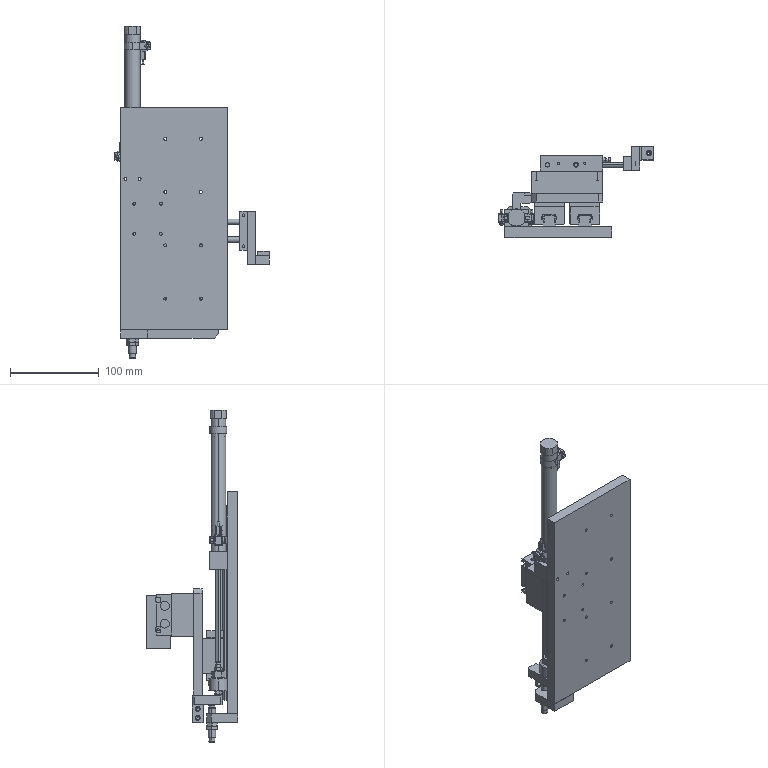Assembly | SolidWorks | mm | 25 component files | 25 solids | 1499 faces | box 174 x 103 x 373.8 mm | volume 833645 mm3 | plane 741 | cylinder 632 | cone 110 | torus 12 | sphere 4 | commonest cylinder face diameters 0.6 x100 0.7 x48 4.5 x44 2 x40 8 x36 2.862 x32 3.3 x28 3 x28
Bill of materials:
F-YBC_SHR28_R_b | 2 |  | Rectangular block with a stepped outline and a profiled channel along its length on one face. The channel has rounded, lobed side recesses. A small cylindrical pin with a rounded end sticks out from one end face.
F-YBCJ2_NTJ-015A | 1 |  | Hexagonal prism with a central round through-bore. The corners are chamfered on both faces, which gives curved edges on the side faces.
F-YBCJ2RKA16-125_ROD | 1 |  | Long, thin straight pin with a thin flat disc head at one end. At the other end it steps down through a short neck to a smaller-diameter tip.
F-YBC_SHR28_220_r | 2 |  | Long straight bar with a constant cross-section. The section has a rounded groove along each side near the top and chamfered or stepped lower corners. A row of four evenly spaced through-holes runs along the bar, passing between the top and bottom faces.
F-YBXCXSM10-15-Z73L_CXSSwitches(Z73) | 2 |  | Long rectangular bar with a plain cylindrical rod sticking out from one end, in line with the bar's length. The bar's cross-section has angled steps or shoulders and a small raised strip on one side.
F-YBXCXSM10-15-Z73L_cyl_cxs(CXS10-15) | 1 |  | Rectangular block with several holes. The top face has two counterbored holes and two small holes. A large side face has two through-holes. One end face has two notched slots with lips at their openings and two round holes. A double-hex fitting with a narrower neck sticks out from that end face.
F-YBXCXSM10-15-Z73L_pr_cxs(PR_CXS_10-15) | 1 |  | Rectangular block with two parallel round rods sticking out from one face. Each rod ends in a short, larger-diameter round head. The block has round holes in two of its faces.
LSDH-6-025 | 1 |  | Thin rectangular plate with chamfered corners and many through-holes: a pair of larger holes near each long edge at one end, two rows of four holes in the middle, and three small holes near the other end.
LSDH-6-026 | 1 |  | L-shaped block: a tall rectangular upright with two through-holes in one face, and a short rectangular foot at its base extending to one side. The foot has one hole in its top face.
LSDH-6-027 | 1 |  | Solid rectangular block. One large face has four through-holes near its corners and two small blind holes on the centreline. The other faces have no visible features.
F-YBJB20-5-080(0) | 1 |  | Stepped turned part, from top to bottom: a hex section with a central blind hole, a large cylinder with a chamfered top edge, a smaller hex section, and a small cylindrical pin with a neck or groove and a chamfered end.
8 | 1 |  | Long cylinder that steps down to a slightly smaller diameter at each end. It has a small central bore at one end and a small notch in the rim at the other end.
8 | 2 |  | Low-profile hexagonal ring shaped like a nut: a flat hex prism with a large central round bore and chamfered/rounded edges at the corners on both faces.
0806 | 1 |  | Solid stepped cylindrical pin: a short, larger-diameter cylindrical base with a longer, smaller-diameter coaxial shaft, both ends flat.
LSDH-4-030 | 1 |  | Thick rectangular, nearly square block with one round through-hole that is slightly off center.
LSDH-6-024 | 1 |  | Thin flat rectangular plate with an irregular pattern of 14 small round through-holes, mostly arranged in pairs.
LSDH-6-028 | 1 |  | L-shaped bracket block: an L-shaped plan form with chamfered outer corners, one vertical through-hole near the end of one arm, and a taller leg at the corner with two parallel horizontal through-holes.
LSDH-6-029 | 1 |  | Thick rectangular block with two chamfered corners on one edge, one larger round through-hole near the chamfered edge, and two smaller round through-holes near the opposite edge.
Mates:
1. coincident | LSDH-6-024-1 face at (319.305, 292.175, 189.479) dir (0, 1, 0) | F-YBCNS_1_1394078242-1/F-YBC_SHR28_220_r-1 face at (302.305, 292.175, 299.479) dir (0, -1, 0)
2. concentric | LSDH-6-024-1 face at (309.305, 292.175, 279.479) dir (0, 1, 0) r 1.65 | F-YBCNS_1_1394078242-1/F-YBC_SHR28_220_r-1 face at (309.305, 292.175, 279.479) dir (0, 1, 0) r 2.25
3. concentric | LSDH-6-024-1 face at (309.305, 292.175, 99.479) dir (0, 1, 0) r 1.65 | F-YBCNS_1_1394078242-1/F-YBC_SHR28_220_r-1 face at (309.305, 292.175, 99.479) dir (0, 1, 0) r 2.25
4. coincident | F-YBCNS_1_1394078242-1/F-YBC_SHR28_220_r-1 face at (314.801, 305.175, 299.479) dir (0, 1, 0) | F-YBCNS_1_1394078242-2/F-YBC_SHR28_220_r-1 face at (354.801, 305.175, 299.479) dir (0, 1, 0)
5. concentric | LSDH-6-024-1 face at (349.305, 292.175, 279.479) dir (0, 1, 0) r 1.65 | F-YBCNS_1_1394078242-2/F-YBC_SHR28_220_r-1 face at (349.305, 292.175, 279.479) dir (0, 1, 0) r 2.25
6. concentric | LSDH-6-024-1 face at (349.305, 292.175, 99.479) dir (0, 1, 0) r 1.65 | F-YBCNS_1_1394078242-2/F-YBC_SHR28_220_r-1 face at (349.305, 292.175, 99.479) dir (0, 1, 0) r 2.25
7. coincident | assembly face at (118.251, 187.005, 82.79) dir (0, 0, -1) | assembly face at (178.251, 187.005, 82.79) dir (0, 0, -1)
8. coincident | F-YBCNS_1_1394078242-1/F-YBC_SHR28_220_r-1 face at (314.805, 297, 299.479) dir (1, 0, 0) | F-YBC_SHR28_R_b-1 face at (314.805, 299.972, 149.729) dir (-1, 0, 0)
9. coincident | F-YBC_SHR28_R_b-1 face at (314.805, 320.175, 110.229) dir (0, 1, 0) | F-YBC_SHR28_R_b-2 face at (354.805, 320.175, 110.229) dir (0, 1, 0)
10. coincident | F-YBCNS_1_1394078242-2/F-YBC_SHR28_220_r-1 face at (343.805, 299.972, 299.479) dir (-1, 0, 0) | F-YBC_SHR28_R_b-2 face at (343.805, 297, 149.729) dir (1, 0, 0)
11. coincident | F-YBC_SHR28_R_b-1 face at (309.305, 292.175, 102.029) dir (0, 0, -1) | F-YBC_SHR28_R_b-2 face at (349.305, 292.175, 102.029) dir (0, 0, -1)
12. coincident | F-YBC_SHR28_R_b-1 face at (314.805, 320.175, 110.229) dir (0, 1, 0) | F-YBExport-1-1/LSDH-6-025-1 face at (329.305, 320.175, 129.979) dir (0, -1, 0)
13. parallel | LSDH-6-024-1 face at (379.305, 292.175, 64.479) dir (1, 0, 0) | F-YBExport-1-1/LSDH-6-025-1 face at (289.305, 330.175, 204.979) dir (-1, 0, 0)
14. concentric | F-YBC_SHR28_R_b-1 face at (296.305, 320.175, 142.979) dir (0, -1, 0) r 1.621 | F-YBExport-1-1/LSDH-6-025-1 face at (296.305, 330.175, 142.979) dir (0, 1, 0) r 2.25
15. concentric | F-YBC_SHR28_R_b-1 face at (322.305, 320.175, 116.979) dir (0, -1, 0) r 1.621 | F-YBExport-1-1/LSDH-6-025-1 face at (322.305, 330.175, 116.979) dir (0, 1, 0) r 2.25
16. concentric | F-YBC_SHR28_R_b-2 face at (336.305, 320.175, 116.979) dir (0, -1, 0) r 1.621 | F-YBExport-1-1/LSDH-6-025-1 face at (336.305, 330.175, 116.979) dir (0, 1, 0) r 2.25
17. concentric | F-YBC_SHR28_R_b-2 face at (362.305, 320.175, 142.979) dir (0, -1, 0) r 1.621 | F-YBExport-1-1/LSDH-6-025-1 face at (362.305, 330.175, 142.979) dir (0, 1, 0) r 2.25
18. coincident | LSDH-6-024-1 face at (319.305, 292.175, 189.479) dir (0, 1, 0) | F-YBCDJ2RKA16-125-M9NL(0_0_0)-1/F-YBCJ2RKA16-125-M9N(0_0)_BODY-1 face at (259.305, 292.175, 246.979) dir (0, -1, 0)
19. parallel | LSDH-6-024-1 face at (259.305, 292.175, 64.479) dir (-1, 0, 0) | F-YBCDJ2RKA16-125-M9NL(0_0_0)-1/F-YBCJ2RKA16-125-M9N(0_0)_BODY-1 face at (285.305, 292.175, 246.979) dir (1, 0, 0)
20. concentric | assembly face at (58.85, 497.004, 336.1) dir (0, 0, -1) r 2.5 | F-YBJB20-5-080(0)-1 face at (272.305, 302.175, 112.479) dir (0, 0, 1) r 2.5
21. concentric | F-YBCDJ2RKA16-125-M9NL(0_0_0)-1/F-YBCJ2RKA16-125-M9N(0_0)_BODY-1 face at (272.305, 302.175, 276.479) dir (0, 0, -1) r 8 | F-YBCJ2RKA16-125_ROD-1 face at (272.305, 302.175, 275.979) dir (0, 0, -1) r 8
22. distance | F-YBCJ2RKA16-125_ROD-1 face at (272.305, 310.175, 275.979) dir (0, 0, 1) | F-YBCDJ2RKA16-125-M9NL(0_0_0)-1/F-YBCJ2RKA16-125-M9N(0_0)_BODY-1 face at (272.305, 310.175, 376.979) dir (0, 0, -1)
23. concentric | F-YBJB20-5-080(0)-1 face at (272.305, 302.175, 112.479) dir (0, 0, 1) r 2.5 | F-YBCJ2RKA16-125_ROD-1 face at (272.305, 302.175, 275.979) dir (0, 0, -1) r 2.5
24. distance | F-YBCJ2RKA16-125_ROD-1 face at (272.305, 304.675, 120.479) dir (0, 0, 1) | F-YBJB20-5-080(0)-1 face at (272.305, 308.675, 112.479) dir (0, 0, 1)
25. concentric | F-YBCJ2RKA16-125_ROD-1 face at (272.305, 302.175, 275.979) dir (0, 0, -1) r 2.5 | F-YBCJ2_NTJ-015A-1 face at (272.305, 302.175, 112.479) dir (0, 0, 1) r 2.5
26. coincident | F-YBJB20-5-080(0)-1 face at (272.305, 308.675, 112.479) dir (0, 0, 1) | F-YBCJ2_NTJ-015A-1 face at (272.305, 302.175, 112.479) dir (0, 0, -1)
27. concentric | LSDH-6-024-1 face at (264.305, 292.175, 234.479) dir (0, 1, 0) r 1.65 | F-YBCDJ2RKA16-125-M9NL(0_0_0)-1/F-YBCJ2RKA16-125-M9N(0_0)_BODY-1 face at (264.305, 312.175, 234.479) dir (0, 1, 0) r 2.25
28. concentric | LSDH-6-024-1 face at (280.305, 292.175, 234.479) dir (0, 1, 0) r 1.65 | F-YBCDJ2RKA16-125-M9NL(0_0_0)-1/F-YBCJ2RKA16-125-M9N(0_0)_BODY-1 face at (280.305, 312.175, 234.479) dir (0, 1, 0) r 2.25
29. coincident | F-YBExport-1-1/LSDH-6-025-1 face at (289.305, 330.175, 204.979) dir (-1, 0, 0) | LSDH-6-028-1 face at (289.305, 319.175, 54.479) dir (1, 0, 0)
30. concentric | F-YBJB20-5-080(0)-1 face at (272.305, 302.175, 112.479) dir (0, 0, -1) r 2.5 | LSDH-6-028-1 face at (272.305, 302.175, 84.479) dir (0, 0, 1) r 2.5
31. coincident | F-YBJB20-5-080(0)-1 face at (272.305, 304.675, 84.479) dir (0, 0, 1) | LSDH-6-028-1 face at (289.305, 319.175, 84.479) dir (0, 0, 1)
32. concentric | LSDH-6-024-1 face at (266.805, 286.175, 64.479) dir (0, 0, -1) r 2.1 | LSDH-6-029-1 face at (266.805, 286.175, 54.479) dir (0, 0, -1) r 2.25
33. concentric | LSDH-6-024-1 face at (281.805, 286.175, 64.479) dir (0, 0, -1) r 2.1 | LSDH-6-029-1 face at (281.805, 286.175, 54.479) dir (0, 0, -1) r 2.25
34. coincident | LSDH-6-024-1 face at (379.305, 292.175, 64.479) dir (0, 0, -1) | LSDH-6-029-1 face at (274.305, 297.675, 64.479) dir (0, 0, 1)
35. coincident | F-YBXFJFA-RB0806-1/F-YBXFJFA-RB0806_Rb-Nut-1 face at (282.697, 315.175, 54.479) dir (0, 0, 1) | LSDH-6-029-1 face at (274.305, 297.675, 54.479) dir (0, 0, -1)
36. concentric | F-YBXFJFA-RB0806-1/F-YBXFJFA-RB0806_Rb-Body-1 face at (272.305, 309.175, 73.479) dir (0, 0, -1) r 4 | LSDH-6-029-1 face at (272.305, 309.175, 64.479) dir (0, 0, 1) r 4
37. coincident | F-YBExport-1-1/LSDH-6-026-1 face at (436.305, 383.175, 147.979) dir (0, 0, 1) | LSDH-4-030-1 face at (424.805, 375.175, 147.979) dir (0, 0, -1)
38. concentric | F-YBExport-1-1/LSDH-6-026-1 face at (421.305, 375.175, 147.979) dir (0, 0, 1) r 1.25 | LSDH-4-030-1 face at (421.305, 375.175, 152.979) dir (0, 0, 1) r 1.7
39. concentric | F-YBExport-1-1/LSDH-6-025-1 face at (289.305, 325.175, 69.979) dir (-1, 0, 0) r 2.1 | LSDH-6-028-1 face at (279.305, 325.175, 69.979) dir (-1, 0, 0) r 2.75
40. concentric | F-YBExport-1-1/LSDH-6-025-1 face at (289.305, 325.175, 59.979) dir (-1, 0, 0) r 2.1 | LSDH-6-028-1 face at (279.305, 325.175, 59.979) dir (-1, 0, 0) r 2.75
41. coincident | F-YBXCXSM10-15-Z73L-1/F-YBXCXSM10-15-Z73L_pr_cxs(PR_CXS_10-15)-1 face at (-25.879, -54.55, 35.136) dir (0, -1, 0) | LSDH-6-026-1 face at (-69.879, -54.55, 47.136) dir (0, 1, 0)
42. coincident | LSDH-6-025-1 face at (-1.879, 17.45, -5.864) dir (0, 0, 1) | LSDH-6-027-1 face at (-47.879, 17.45, -5.864) dir (0, 0, -1)
43. coincident | LSDH-6-025-1 face at (-1.879, 17.45, -5.864) dir (0, 0, 1) | LSDH-6-027-1 face at (-47.879, 17.45, -5.864) dir (0, 0, -1)
44. concentric | F-YBXCXSM10-15-Z73L-1/F-YBXCXSM10-15-Z73L_cyl_cxs(CXS10-15)-1 face at (-47.879, 27.45, 14.629) dir (0, 0, -1) r 1.7 | LSDH-6-027-1 face at (-47.879, 27.45, 19.136) dir (0, 0, 1) r 1.25
45. coincident | F-YBXCXSM10-15-Z73L-1/F-YBXCXSM10-15-Z73L_cyl_cxs(CXS10-15)-1 face at (-24.879, 47.45, 19.136) dir (0, 0, -1) | LSDH-6-027-1 face at (-47.879, 17.45, 19.136) dir (0, 0, 1)
46. concentric | F-YBXCXSM10-15-Z73L-1/F-YBXCXSM10-15-Z73L_cyl_cxs(CXS10-15)-1 face at (-47.879, -2.55, 14.629) dir (0, 0, -1) r 1.7 | LSDH-6-027-1 face at (-47.879, -2.55, 19.136) dir (0, 0, 1) r 1.25
47. concentric | F-YBXCXSM10-15-Z73L-1/F-YBXCXSM10-15-Z73L_pr_cxs(PR_CXS_10-15)-1 face at (-30.379, -54.55, 27.636) dir (0, 1, 0) r 2 | LSDH-6-026-1 face at (-30.379, -64.55, 27.636) dir (0, -1, 0) r 4
48. concentric | F-YBXCXSM10-15-Z73L-1/F-YBXCXSM10-15-Z73L_pr_cxs(PR_CXS_10-15)-1 face at (-65.379, -54.55, 27.636) dir (0, 1, 0) r 2 | LSDH-6-026-1 face at (-65.379, -64.55, 27.636) dir (0, -1, 0) r 4
49. concentric | LSDH-6-025-1 face at (-65.879, 51.45, -5.864) dir (0, 0, 1) r 2.1 | LSDH-6-027-1 face at (-65.879, 51.45, 14.136) dir (0, 0, 1) r 2.75
50. concentric | LSDH-6-025-1 face at (-29.879, 51.45, -5.864) dir (0, 0, 1) r 2.1 | LSDH-6-027-1 face at (-29.879, 51.45, 14.136) dir (0, 0, 1) r 2.75
51. concentric | F-YBXCXSM10-15-Z73L_cyl_cxs(CXS10-15)-1 face at (10, 0, -10) dir (0, 0, 1) r 3.05 | F-YBXCXSM10-15-Z73L_pr_cxs(PR_CXS_10-15)-1 face at (10, 0, -15) dir (0, 0, 1) r 3
52. concentric | F-YBXCXSM10-15-Z73L_cyl_cxs(CXS10-15)-1 face at (-10, 0, -10) dir (0, 0, 1) r 3.05 | F-YBXCXSM10-15-Z73L_pr_cxs(PR_CXS_10-15)-1 face at (-10, 0, -15) dir (0, 0, 1) r 3
53. distance | F-YBXCXSM10-15-Z73L_pr_cxs(PR_CXS_10-15)-1 face at (10, 0, -15) dir (0, 0, -1) | F-YBXCXSM10-15-Z73L_cyl_cxs(CXS10-15)-1 face at (10, 0, -30) dir (0, 0, 1)
54. concentric | F-YBXFJFA-RB0806_Rb-Body-1 face at (0, 0, 5.4) dir (0, 0, 1) r 1.4 | F-YBXFJFA-RB0806_Rb-Rod-1 face at (0, 0, 5.4) dir (0, 0, 1) r 2.4
55. concentric | F-YBXFJFA-RB0806_Rb-Body-1 face at (0, 0, 20.4) dir (0, 0, -1) r 4 | F-YBXFJFA-RB0806_Rb-Nut-1 face at (0, 0, 1.4) dir (0, 0, -1) r 4
56. distance | F-YBXFJFA-RB0806_Rb-Nut-1 face at (10.392, 6, 1.4) dir (0, 0, 1) | F-YBXFJFA-RB0806 plane at (0, 0, 0) dir (0, 0, 1)
57. parallel | F-YBXFJFA-RB0806_Rb-Nut-1 face at (3.464, 6, 1.4) dir (0, 1, 0) | F-YBXFJFA-RB0806 plane at (0, 0, 0) dir (0, 1, 0)
58. concentric | F-YBXFJFA-RB0806_Rb-Body-1 face at (0, 0, 20.4) dir (0, 0, -1) r 4 | F-YBXFJFA-RB0806_Rb-Nut-2 face at (0, 0, -2.6) dir (0, 0, -1) r 4
59. distance | F-YBXFJFA-RB0806_Rb-Nut-1 face at (10.392, 6, -2.6) dir (0, 0, -1) | F-YBXFJFA-RB0806_Rb-Nut-2 face at (10.392, 6, -2.6) dir (0, 0, 1)
60. parallel | F-YBXFJFA-RB0806_Rb-Nut-2 face at (3.464, 6, -2.6) dir (0, 1, 0) | F-YBXFJFA-RB0806 plane at (0, 0, 0) dir (0, 1, 0)
61. coincident | F-YBXFJFA-RB0806_Rb-Body-1 face at (0, 0, 5.4) dir (0, 0, 1) | F-YBXFJFA-RB0806_Rb-Rod-1 face at (0, 0, 5.4) dir (0, 0, -1)